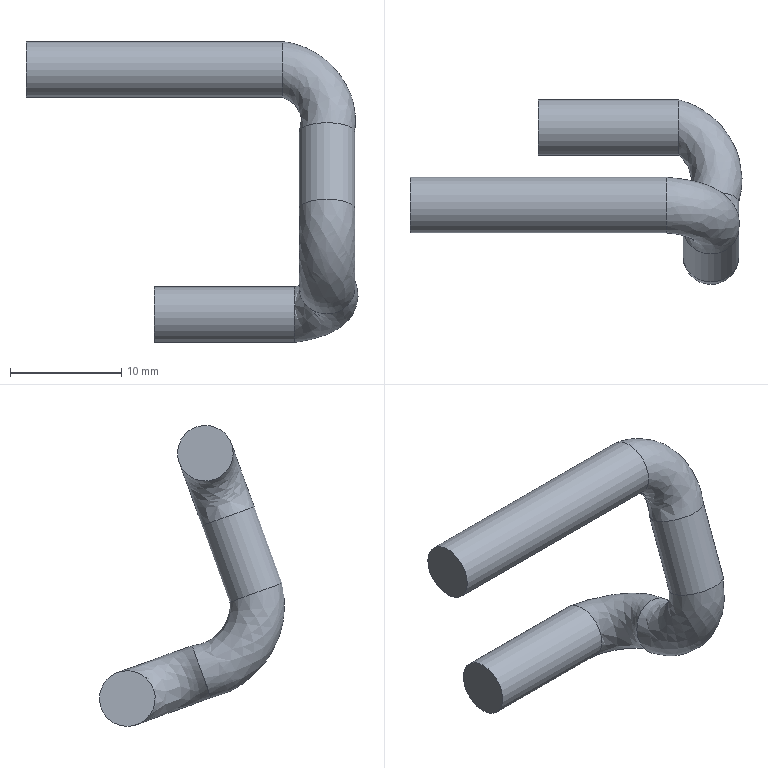Component | NX | HOSE | 2 solids | 10 faces | box 29.94 x 16.61 x 27 mm | volume 1335 mm3 | plane 4 | cylinder 3 | other 3 | commonest cylinder face diameters 5 x3
STEP:
#1=CARTESIAN_POINT('',(0.,0.,0.));
#2=DIRECTION('',(0.,0.,1.));
#3=DIRECTION('',(1.,0.,0.));
#4=AXIS2_PLACEMENT_3D('',#1,#2,#3);
#5=CARTESIAN_POINT('',(84.825,2.35,-26.852));
#6=VERTEX_POINT('',#5);
#7=CARTESIAN_POINT('',(84.825,0.,-26.));
#8=DIRECTION('',(1.,-0.,0.));
#9=DIRECTION('',(0.,0.9402,-0.3406));
#10=AXIS2_PLACEMENT_3D('',#7,#8,#9);
#11=CIRCLE('',#10,2.5);
#12=CARTESIAN_POINT('',(84.825,0.,-26.));
#13=DIRECTION('',(-1.,0.,0.));
#14=DIRECTION('',(0.,0.3406,0.9402));
#15=AXIS2_PLACEMENT_3D('',#12,#13,#14);
#16=CYLINDRICAL_SURFACE('',#15,2.5);
#17=CARTESIAN_POINT('',(7.854,0.));
#18=DIRECTION('',(-1.,0.));
#19=VECTOR('',#18,1.);
#20=LINE('',#17,#19);
#21=(GEOMETRIC_REPRESENTATION_CONTEXT(2)PARAMETRIC_REPRESENTATION_CONTEXT()REPRESENTATION_CONTEXT('',''));
#22=DEFINITIONAL_REPRESENTATION('',(#20),#21);
#23=PCURVE('',#16,#22);
#24=CARTESIAN_POINT('',(84.825,0.,-26.));
#25=DIRECTION('',(1.,-0.,0.));
#26=DIRECTION('',(0.,0.9402,-0.3406));
#27=AXIS2_PLACEMENT_3D('',#24,#25,#26);
#28=CIRCLE('',#27,2.5);
#29=CARTESIAN_POINT('',(82.75,-4.701,-24.297));
#30=DIRECTION('',(0.,-0.3406,-0.9402));
#31=AXIS1_PLACEMENT('',#29,#30);
#32=SURFACE_OF_REVOLUTION('',#28,#31);
#33=CARTESIAN_POINT('',(6.283,0.));
#34=DIRECTION('',(0.,1.));
#35=VECTOR('',#34,1.);
#36=LINE('',#33,#35);
#37=(GEOMETRIC_REPRESENTATION_CONTEXT(2)PARAMETRIC_REPRESENTATION_CONTEXT()REPRESENTATION_CONTEXT('',''));
#38=DEFINITIONAL_REPRESENTATION('',(#36),#37);
#39=PCURVE('',#32,#38);
#40=SURFACE_CURVE('',#11,(#23,#39),.PCURVE_S1.);
#41=EDGE_CURVE('',#6,#6,#40,.T.);
#42=ORIENTED_EDGE('',*,*,#41,.F.);
#43=CARTESIAN_POINT('',(72.25,2.35,-26.852));
#44=VERTEX_POINT('',#43);
#45=CARTESIAN_POINT('',(84.825,2.35,-26.852));
#46=CARTESIAN_POINT('',(72.25,2.35,-26.852));
#47=B_SPLINE_CURVE_WITH_KNOTS('',1,(#45,#46),.UNSPECIFIED.,.F.,.F.,(2,2),(0.,12.575),.PIECEWISE_BEZIER_KNOTS.);
#48=CARTESIAN_POINT('',(7.854,0.));
#49=DIRECTION('',(0.,1.));
#50=VECTOR('',#49,1.);
#51=LINE('',#48,#50);
#52=(GEOMETRIC_REPRESENTATION_CONTEXT(2)PARAMETRIC_REPRESENTATION_CONTEXT()REPRESENTATION_CONTEXT('',''));
#53=DEFINITIONAL_REPRESENTATION('',(#51),#52);
#54=PCURVE('',#16,#53);
#55=CARTESIAN_POINT('',(1.571,0.));
#56=DIRECTION('',(0.,1.));
#57=VECTOR('',#56,1.);
#58=LINE('',#55,#57);
#59=(GEOMETRIC_REPRESENTATION_CONTEXT(2)PARAMETRIC_REPRESENTATION_CONTEXT()REPRESENTATION_CONTEXT('',''));
#60=DEFINITIONAL_REPRESENTATION('',(#58),#59);
#61=PCURVE('',#16,#60);
#62=SEAM_CURVE('',#47,(#54,#61),.PCURVE_S1.);
#63=EDGE_CURVE('',#6,#44,#62,.T.);
#64=ORIENTED_EDGE('',*,*,#63,.T.);
#65=CARTESIAN_POINT('',(72.25,0.,-26.));
#66=DIRECTION('',(1.,-0.,0.));
#67=DIRECTION('',(0.,0.9402,-0.3406));
#68=AXIS2_PLACEMENT_3D('',#65,#66,#67);
#69=CIRCLE('',#68,2.5);
#70=CARTESIAN_POINT('',(7.854,12.575));
#71=DIRECTION('',(-1.,0.));
#72=VECTOR('',#71,1.);
#73=LINE('',#70,#72);
#74=(GEOMETRIC_REPRESENTATION_CONTEXT(2)PARAMETRIC_REPRESENTATION_CONTEXT()REPRESENTATION_CONTEXT('',''));
#75=DEFINITIONAL_REPRESENTATION('',(#73),#74);
#76=PCURVE('',#16,#75);
#77=CARTESIAN_POINT('',(72.25,0.,-26.));
#78=DIRECTION('',(1.,-0.,0.));
#79=DIRECTION('',(0.,-0.3406,-0.9402));
#80=AXIS2_PLACEMENT_3D('',#77,#78,#79);
#81=PLANE('',#80);
#82=CARTESIAN_POINT('',(0.,0.));
#83=DIRECTION('',(0.,1.));
#84=AXIS2_PLACEMENT_2D('',#82,#83);
#85=CIRCLE('',#84,2.5);
#86=(GEOMETRIC_REPRESENTATION_CONTEXT(2)PARAMETRIC_REPRESENTATION_CONTEXT()REPRESENTATION_CONTEXT('',''));
#87=DEFINITIONAL_REPRESENTATION('',(#85),#86);
#88=PCURVE('',#81,#87);
#89=SURFACE_CURVE('',#69,(#76,#88),.PCURVE_S1.);
#90=EDGE_CURVE('',#44,#44,#89,.T.);
#91=ORIENTED_EDGE('',*,*,#90,.T.);
#92=ORIENTED_EDGE('',*,*,#63,.F.);
#93=EDGE_LOOP('',(#42,#64,#91,#92));
#94=FACE_BOUND('',#93,.T.);
#95=ADVANCED_FACE('',(#94),#16,.T.);
#96=ORIENTED_EDGE('',*,*,#41,.F.);
#97=CARTESIAN_POINT('',(90.25,-6.652,-23.59));
#98=VERTEX_POINT('',#97);
#99=CARTESIAN_POINT('',(84.825,2.35,-26.852));
#100=CARTESIAN_POINT('',(86.83,1.829,-26.663));
#101=CARTESIAN_POINT('',(88.607,0.7215,-26.261));
#102=CARTESIAN_POINT('',(89.95,-0.8659,-25.686));
#103=CARTESIAN_POINT('',(90.708,-2.765,-24.998));
#104=CARTESIAN_POINT('',(90.805,-4.767,-24.273));
#105=CARTESIAN_POINT('',(90.25,-6.652,-23.59));
#106=(BOUNDED_CURVE()B_SPLINE_CURVE(6,(#99,#100,#101,#102,#103,#104,#105),.UNSPECIFIED.,.F.,.F.)B_SPLINE_CURVE_WITH_KNOTS((7,7),(0.,1.571),.PIECEWISE_BEZIER_KNOTS.)CURVE()GEOMETRIC_REPRESENTATION_ITEM()RATIONAL_B_SPLINE_CURVE((1.031,1.01,0.9979,0.994,0.9979,1.01,1.031))REPRESENTATION_ITEM(''));
#107=CARTESIAN_POINT('',(6.283,0.));
#108=DIRECTION('',(1.,0.));
#109=VECTOR('',#108,1.);
#110=LINE('',#107,#109);
#111=(GEOMETRIC_REPRESENTATION_CONTEXT(2)PARAMETRIC_REPRESENTATION_CONTEXT()REPRESENTATION_CONTEXT('',''));
#112=DEFINITIONAL_REPRESENTATION('',(#110),#111);
#113=PCURVE('',#32,#112);
#114=CARTESIAN_POINT('',(6.283,6.283));
#115=DIRECTION('',(1.,0.));
#116=VECTOR('',#115,1.);
#117=LINE('',#114,#116);
#118=(GEOMETRIC_REPRESENTATION_CONTEXT(2)PARAMETRIC_REPRESENTATION_CONTEXT()REPRESENTATION_CONTEXT('',''));
#119=DEFINITIONAL_REPRESENTATION('',(#117),#118);
#120=PCURVE('',#32,#119);
#121=SEAM_CURVE('',#106,(#113,#120),.PCURVE_S1.);
#122=EDGE_CURVE('',#6,#98,#121,.T.);
#123=ORIENTED_EDGE('',*,*,#122,.T.);
#124=CARTESIAN_POINT('',(87.75,-6.652,-23.59));
#125=DIRECTION('',(0.,-0.9402,0.3406));
#126=DIRECTION('',(1.,0.,0.));
#127=AXIS2_PLACEMENT_3D('',#124,#125,#126);
#128=CIRCLE('',#127,2.5);
#129=CARTESIAN_POINT('',(7.854,0.));
#130=DIRECTION('',(0.,1.));
#131=VECTOR('',#130,1.);
#132=LINE('',#129,#131);
#133=(GEOMETRIC_REPRESENTATION_CONTEXT(2)PARAMETRIC_REPRESENTATION_CONTEXT()REPRESENTATION_CONTEXT('',''));
#134=DEFINITIONAL_REPRESENTATION('',(#132),#133);
#135=PCURVE('',#32,#134);
#136=CARTESIAN_POINT('',(87.75,-6.652,-23.59));
#137=DIRECTION('',(0.,-0.9402,0.3406));
#138=DIRECTION('',(0.,-0.3406,-0.9402));
#139=AXIS2_PLACEMENT_3D('',#136,#137,#138);
#140=PLANE('',#139);
#141=CARTESIAN_POINT('',(0.,0.));
#142=DIRECTION('',(0.,1.));
#143=AXIS2_PLACEMENT_2D('',#141,#142);
#144=CIRCLE('',#143,2.5);
#145=(GEOMETRIC_REPRESENTATION_CONTEXT(2)PARAMETRIC_REPRESENTATION_CONTEXT()REPRESENTATION_CONTEXT('',''));
#146=DEFINITIONAL_REPRESENTATION('',(#144),#145);
#147=PCURVE('',#140,#146);
#148=SURFACE_CURVE('',#128,(#135,#147),.PCURVE_S1.);
#149=EDGE_CURVE('',#98,#98,#148,.T.);
#150=ORIENTED_EDGE('',*,*,#149,.T.);
#151=ORIENTED_EDGE('',*,*,#122,.F.);
#152=EDGE_LOOP('',(#96,#123,#150,#151));
#153=FACE_BOUND('',#152,.F.);
#154=ADVANCED_FACE('',(#153),#32,.F.);
#155=ORIENTED_EDGE('',*,*,#90,.F.);
#156=EDGE_LOOP('',(#155));
#157=FACE_BOUND('',#156,.T.);
#158=ADVANCED_FACE('',(#157),#81,.F.);
#159=ORIENTED_EDGE('',*,*,#149,.T.);
#160=EDGE_LOOP('',(#159));
#161=FACE_BOUND('',#160,.T.);
#162=ADVANCED_FACE('',(#161),#140,.T.);
#163=CLOSED_SHELL('',(#95,#154,#158,#162));
#164=MANIFOLD_SOLID_BREP('',#163);
#165=(LENGTH_UNIT()NAMED_UNIT(*)SI_UNIT(.MILLI.,.METRE.));
#166=UNCERTAINTY_MEASURE_WITH_UNIT(LENGTH_MEASURE(0.00001),#165,'','');
#167=(NAMED_UNIT(*)PLANE_ANGLE_UNIT()SI_UNIT($,.RADIAN.));
#168=(NAMED_UNIT(*)SI_UNIT($,.STERADIAN.)SOLID_ANGLE_UNIT());
#169=(GEOMETRIC_REPRESENTATION_CONTEXT(3)GLOBAL_UNCERTAINTY_ASSIGNED_CONTEXT((#166))GLOBAL_UNIT_ASSIGNED_CONTEXT((#165,#167,#168))REPRESENTATION_CONTEXT('',''));
#170=ADVANCED_BREP_SHAPE_REPRESENTATION('',(#4,#164),#169);
#171=CARTESIAN_POINT('',(0.,0.,0.));
#172=DIRECTION('',(0.,0.,1.));
#173=DIRECTION('',(1.,0.,0.));
#174=AXIS2_PLACEMENT_3D('',#171,#172,#173);
#175=CARTESIAN_POINT('',(0.,0.,0.));
#176=DIRECTION('',(0.,0.,1.));
#177=DIRECTION('',(1.,0.,0.));
#178=AXIS2_PLACEMENT_3D('',#175,#176,#177);
#179=(LENGTH_UNIT()NAMED_UNIT(*)SI_UNIT(.MILLI.,.METRE.));
#180=UNCERTAINTY_MEASURE_WITH_UNIT(LENGTH_MEASURE(0.00001),#179,'','');
#181=(NAMED_UNIT(*)PLANE_ANGLE_UNIT()SI_UNIT($,.RADIAN.));
#182=(NAMED_UNIT(*)SI_UNIT($,.STERADIAN.)SOLID_ANGLE_UNIT());
#183=(GEOMETRIC_REPRESENTATION_CONTEXT(3)GLOBAL_UNCERTAINTY_ASSIGNED_CONTEXT((#180))GLOBAL_UNIT_ASSIGNED_CONTEXT((#179,#181,#182))REPRESENTATION_CONTEXT('',''));
#184=SHAPE_REPRESENTATION('',(#4,#174,#178),#183);
#185=ITEM_DEFINED_TRANSFORMATION('','',#4,#174);
#186=(REPRESENTATION_RELATIONSHIP('','',#170,#184)REPRESENTATION_RELATIONSHIP_WITH_TRANSFORMATION(#185)SHAPE_REPRESENTATION_RELATIONSHIP());
#187=CARTESIAN_POINT('',(83.75,-6.148,-1.65));
#188=VERTEX_POINT('',#187);
#189=CARTESIAN_POINT('',(83.75,-7.,-4.));
#190=DIRECTION('',(-1.,-0.,0.));
#191=DIRECTION('',(0.,0.3406,0.9402));
#192=AXIS2_PLACEMENT_3D('',#189,#190,#191);
#193=CIRCLE('',#192,2.5);
#194=CARTESIAN_POINT('',(83.75,-7.,-4.));
#195=DIRECTION('',(-1.,0.,0.));
#196=DIRECTION('',(0.,0.3406,0.9402));
#197=AXIS2_PLACEMENT_3D('',#194,#195,#196);
#198=CYLINDRICAL_SURFACE('',#197,2.5);
#199=CARTESIAN_POINT('',(0.,0.));
#200=DIRECTION('',(1.,0.));
#201=VECTOR('',#200,1.);
#202=LINE('',#199,#201);
#203=(GEOMETRIC_REPRESENTATION_CONTEXT(2)PARAMETRIC_REPRESENTATION_CONTEXT()REPRESENTATION_CONTEXT('',''));
#204=DEFINITIONAL_REPRESENTATION('',(#202),#203);
#205=PCURVE('',#198,#204);
#206=CARTESIAN_POINT('',(87.75,-9.044,-9.641));
#207=DIRECTION('',(0.,0.3406,0.9402));
#208=DIRECTION('',(1.,-0.,0.));
#209=AXIS2_PLACEMENT_3D('',#206,#207,#208);
#210=CIRCLE('',#209,2.5);
#211=CARTESIAN_POINT('',(82.75,-8.703,-8.701));
#212=DIRECTION('',(0.,-0.9402,0.3406));
#213=AXIS1_PLACEMENT('',#211,#212);
#214=SURFACE_OF_REVOLUTION('',#210,#213);
#215=CARTESIAN_POINT('',(7.854,0.));
#216=DIRECTION('',(0.,1.));
#217=VECTOR('',#216,1.);
#218=LINE('',#215,#217);
#219=(GEOMETRIC_REPRESENTATION_CONTEXT(2)PARAMETRIC_REPRESENTATION_CONTEXT()REPRESENTATION_CONTEXT('',''));
#220=DEFINITIONAL_REPRESENTATION('',(#218),#219);
#221=PCURVE('',#214,#220);
#222=SURFACE_CURVE('',#193,(#205,#221),.PCURVE_S1.);
#223=EDGE_CURVE('',#188,#188,#222,.T.);
#224=ORIENTED_EDGE('',*,*,#223,.T.);
#225=CARTESIAN_POINT('',(60.75,-6.148,-1.65));
#226=VERTEX_POINT('',#225);
#227=CARTESIAN_POINT('',(83.75,-6.148,-1.65));
#228=CARTESIAN_POINT('',(60.75,-6.148,-1.65));
#229=B_SPLINE_CURVE_WITH_KNOTS('',1,(#227,#228),.UNSPECIFIED.,.F.,.F.,(2,2),(0.,23.),.PIECEWISE_BEZIER_KNOTS.);
#230=CARTESIAN_POINT('',(6.283,0.));
#231=DIRECTION('',(0.,1.));
#232=VECTOR('',#231,1.);
#233=LINE('',#230,#232);
#234=(GEOMETRIC_REPRESENTATION_CONTEXT(2)PARAMETRIC_REPRESENTATION_CONTEXT()REPRESENTATION_CONTEXT('',''));
#235=DEFINITIONAL_REPRESENTATION('',(#233),#234);
#236=PCURVE('',#198,#235);
#237=CARTESIAN_POINT('',(0.,0.));
#238=DIRECTION('',(0.,1.));
#239=VECTOR('',#238,1.);
#240=LINE('',#237,#239);
#241=(GEOMETRIC_REPRESENTATION_CONTEXT(2)PARAMETRIC_REPRESENTATION_CONTEXT()REPRESENTATION_CONTEXT('',''));
#242=DEFINITIONAL_REPRESENTATION('',(#240),#241);
#243=PCURVE('',#198,#242);
#244=SEAM_CURVE('',#229,(#236,#243),.PCURVE_S1.);
#245=EDGE_CURVE('',#188,#226,#244,.T.);
#246=ORIENTED_EDGE('',*,*,#245,.T.);
#247=CARTESIAN_POINT('',(60.75,-7.,-4.));
#248=DIRECTION('',(-1.,-0.,0.));
#249=DIRECTION('',(0.,0.3406,0.9402));
#250=AXIS2_PLACEMENT_3D('',#247,#248,#249);
#251=CIRCLE('',#250,2.5);
#252=CARTESIAN_POINT('',(0.,23.));
#253=DIRECTION('',(1.,0.));
#254=VECTOR('',#253,1.);
#255=LINE('',#252,#254);
#256=(GEOMETRIC_REPRESENTATION_CONTEXT(2)PARAMETRIC_REPRESENTATION_CONTEXT()REPRESENTATION_CONTEXT('',''));
#257=DEFINITIONAL_REPRESENTATION('',(#255),#256);
#258=PCURVE('',#198,#257);
#259=CARTESIAN_POINT('',(60.75,-7.,-4.));
#260=DIRECTION('',(-1.,-0.,0.));
#261=DIRECTION('',(0.,-0.9402,0.3406));
#262=AXIS2_PLACEMENT_3D('',#259,#260,#261);
#263=PLANE('',#262);
#264=CARTESIAN_POINT('',(0.,0.));
#265=DIRECTION('',(0.,1.));
#266=AXIS2_PLACEMENT_2D('',#264,#265);
#267=CIRCLE('',#266,2.5);
#268=(GEOMETRIC_REPRESENTATION_CONTEXT(2)PARAMETRIC_REPRESENTATION_CONTEXT()REPRESENTATION_CONTEXT('',''));
#269=DEFINITIONAL_REPRESENTATION('',(#267),#268);
#270=PCURVE('',#263,#269);
#271=SURFACE_CURVE('',#251,(#258,#270),.PCURVE_S1.);
#272=EDGE_CURVE('',#226,#226,#271,.T.);
#273=ORIENTED_EDGE('',*,*,#272,.F.);
#274=ORIENTED_EDGE('',*,*,#245,.F.);
#275=EDGE_LOOP('',(#224,#246,#273,#274));
#276=FACE_BOUND('',#275,.T.);
#277=ADVANCED_FACE('',(#276),#198,.T.);
#278=CARTESIAN_POINT('',(90.25,-9.044,-9.641));
#279=VERTEX_POINT('',#278);
#280=CARTESIAN_POINT('',(87.75,-9.044,-9.641));
#281=DIRECTION('',(0.,0.3406,0.9402));
#282=DIRECTION('',(1.,0.,0.));
#283=AXIS2_PLACEMENT_3D('',#280,#281,#282);
#284=CIRCLE('',#283,2.5);
#285=CARTESIAN_POINT('',(6.283,0.));
#286=DIRECTION('',(0.,1.));
#287=VECTOR('',#286,1.);
#288=LINE('',#285,#287);
#289=(GEOMETRIC_REPRESENTATION_CONTEXT(2)PARAMETRIC_REPRESENTATION_CONTEXT()REPRESENTATION_CONTEXT('',''));
#290=DEFINITIONAL_REPRESENTATION('',(#288),#289);
#291=PCURVE('',#214,#290);
#292=CARTESIAN_POINT('',(87.75,-11.53,-16.505));
#293=DIRECTION('',(0.,0.3406,0.9402));
#294=DIRECTION('',(1.,0.,0.));
#295=AXIS2_PLACEMENT_3D('',#292,#293,#294);
#296=CYLINDRICAL_SURFACE('',#295,2.5);
#297=CARTESIAN_POINT('',(0.,7.3));
#298=DIRECTION('',(1.,0.));
#299=VECTOR('',#298,1.);
#300=LINE('',#297,#299);
#301=(GEOMETRIC_REPRESENTATION_CONTEXT(2)PARAMETRIC_REPRESENTATION_CONTEXT()REPRESENTATION_CONTEXT('',''));
#302=DEFINITIONAL_REPRESENTATION('',(#300),#301);
#303=PCURVE('',#296,#302);
#304=SURFACE_CURVE('',#284,(#291,#303),.PCURVE_S1.);
#305=EDGE_CURVE('',#279,#279,#304,.T.);
#306=ORIENTED_EDGE('',*,*,#305,.F.);
#307=CARTESIAN_POINT('',(90.25,-9.044,-9.641));
#308=CARTESIAN_POINT('',(90.517,-8.361,-7.756));
#309=CARTESIAN_POINT('',(90.14,-7.667,-5.84));
#310=CARTESIAN_POINT('',(89.141,-7.038,-4.106));
#311=CARTESIAN_POINT('',(87.623,-6.545,-2.745));
#312=CARTESIAN_POINT('',(85.755,-6.239,-1.901));
#313=CARTESIAN_POINT('',(83.75,-6.148,-1.65));
#314=(BOUNDED_CURVE()B_SPLINE_CURVE(6,(#307,#308,#309,#310,#311,#312,#313),.UNSPECIFIED.,.F.,.F.)B_SPLINE_CURVE_WITH_KNOTS((7,7),(0.,1.571),.PIECEWISE_BEZIER_KNOTS.)CURVE()GEOMETRIC_REPRESENTATION_ITEM()RATIONAL_B_SPLINE_CURVE((1.031,1.01,0.9979,0.994,0.9979,1.01,1.031))REPRESENTATION_ITEM(''));
#315=CARTESIAN_POINT('',(6.283,0.));
#316=DIRECTION('',(1.,0.));
#317=VECTOR('',#316,1.);
#318=LINE('',#315,#317);
#319=(GEOMETRIC_REPRESENTATION_CONTEXT(2)PARAMETRIC_REPRESENTATION_CONTEXT()REPRESENTATION_CONTEXT('',''));
#320=DEFINITIONAL_REPRESENTATION('',(#318),#319);
#321=PCURVE('',#214,#320);
#322=CARTESIAN_POINT('',(6.283,6.283));
#323=DIRECTION('',(1.,0.));
#324=VECTOR('',#323,1.);
#325=LINE('',#322,#324);
#326=(GEOMETRIC_REPRESENTATION_CONTEXT(2)PARAMETRIC_REPRESENTATION_CONTEXT()REPRESENTATION_CONTEXT('',''));
#327=DEFINITIONAL_REPRESENTATION('',(#325),#326);
#328=PCURVE('',#214,#327);
#329=SEAM_CURVE('',#314,(#321,#328),.PCURVE_S1.);
#330=EDGE_CURVE('',#279,#188,#329,.T.);
#331=ORIENTED_EDGE('',*,*,#330,.T.);
#332=ORIENTED_EDGE('',*,*,#223,.T.);
#333=ORIENTED_EDGE('',*,*,#330,.F.);
#334=EDGE_LOOP('',(#306,#331,#332,#333));
#335=FACE_BOUND('',#334,.F.);
#336=ADVANCED_FACE('',(#335),#214,.F.);
#337=CARTESIAN_POINT('',(90.25,-11.53,-16.505));
#338=VERTEX_POINT('',#337);
#339=CARTESIAN_POINT('',(87.75,-11.53,-16.505));
#340=DIRECTION('',(0.,0.3406,0.9402));
#341=DIRECTION('',(1.,0.,0.));
#342=AXIS2_PLACEMENT_3D('',#339,#340,#341);
#343=CIRCLE('',#342,2.5);
#344=CARTESIAN_POINT('',(0.,0.));
#345=DIRECTION('',(1.,0.));
#346=VECTOR('',#345,1.);
#347=LINE('',#344,#346);
#348=(GEOMETRIC_REPRESENTATION_CONTEXT(2)PARAMETRIC_REPRESENTATION_CONTEXT()REPRESENTATION_CONTEXT('',''));
#349=DEFINITIONAL_REPRESENTATION('',(#347),#348);
#350=PCURVE('',#296,#349);
#351=CARTESIAN_POINT('',(87.75,-11.53,-16.505));
#352=DIRECTION('',(0.,0.3406,0.9402));
#353=DIRECTION('',(1.,-0.,0.));
#354=AXIS2_PLACEMENT_3D('',#351,#352,#353);
#355=CIRCLE('',#354,2.5);
#356=CARTESIAN_POINT('',(87.75,-5.549,-17.608));
#357=DIRECTION('',(1.,0.,0.));
#358=AXIS1_PLACEMENT('',#356,#357);
#359=SURFACE_OF_REVOLUTION('',#355,#358);
#360=CARTESIAN_POINT('',(6.283,0.));
#361=DIRECTION('',(0.,1.));
#362=VECTOR('',#361,1.);
#363=LINE('',#360,#362);
#364=(GEOMETRIC_REPRESENTATION_CONTEXT(2)PARAMETRIC_REPRESENTATION_CONTEXT()REPRESENTATION_CONTEXT('',''));
#365=DEFINITIONAL_REPRESENTATION('',(#363),#364);
#366=PCURVE('',#359,#365);
#367=SURFACE_CURVE('',#343,(#350,#366),.PCURVE_S1.);
#368=EDGE_CURVE('',#338,#338,#367,.T.);
#369=ORIENTED_EDGE('',*,*,#368,.T.);
#370=CARTESIAN_POINT('',(90.25,-11.53,-16.505));
#371=CARTESIAN_POINT('',(90.25,-9.044,-9.641));
#372=B_SPLINE_CURVE_WITH_KNOTS('',1,(#370,#371),.UNSPECIFIED.,.F.,.F.,(2,2),(0.,7.3),.PIECEWISE_BEZIER_KNOTS.);
#373=CARTESIAN_POINT('',(6.283,0.));
#374=DIRECTION('',(0.,1.));
#375=VECTOR('',#374,1.);
#376=LINE('',#373,#375);
#377=(GEOMETRIC_REPRESENTATION_CONTEXT(2)PARAMETRIC_REPRESENTATION_CONTEXT()REPRESENTATION_CONTEXT('',''));
#378=DEFINITIONAL_REPRESENTATION('',(#376),#377);
#379=PCURVE('',#296,#378);
#380=CARTESIAN_POINT('',(0.,0.));
#381=DIRECTION('',(0.,1.));
#382=VECTOR('',#381,1.);
#383=LINE('',#380,#382);
#384=(GEOMETRIC_REPRESENTATION_CONTEXT(2)PARAMETRIC_REPRESENTATION_CONTEXT()REPRESENTATION_CONTEXT('',''));
#385=DEFINITIONAL_REPRESENTATION('',(#383),#384);
#386=PCURVE('',#296,#385);
#387=SEAM_CURVE('',#372,(#379,#386),.PCURVE_S1.);
#388=EDGE_CURVE('',#338,#279,#387,.T.);
#389=ORIENTED_EDGE('',*,*,#388,.T.);
#390=ORIENTED_EDGE('',*,*,#305,.F.);
#391=ORIENTED_EDGE('',*,*,#388,.F.);
#392=EDGE_LOOP('',(#369,#389,#390,#391));
#393=FACE_BOUND('',#392,.T.);
#394=ADVANCED_FACE('',(#393),#296,.T.);
#395=ORIENTED_EDGE('',*,*,#368,.F.);
#396=CARTESIAN_POINT('',(90.25,-6.652,-23.59));
#397=VERTEX_POINT('',#396);
#398=CARTESIAN_POINT('',(90.25,-11.53,-16.505));
#399=CARTESIAN_POINT('',(90.25,-11.825,-18.104));
#400=CARTESIAN_POINT('',(90.25,-11.604,-19.755));
#401=CARTESIAN_POINT('',(90.25,-10.876,-21.276));
#402=CARTESIAN_POINT('',(90.25,-9.715,-22.499));
#403=CARTESIAN_POINT('',(90.25,-8.251,-23.295));
#404=CARTESIAN_POINT('',(90.25,-6.652,-23.59));
#405=(BOUNDED_CURVE()B_SPLINE_CURVE(6,(#398,#399,#400,#401,#402,#403,#404),.UNSPECIFIED.,.F.,.F.)B_SPLINE_CURVE_WITH_KNOTS((7,7),(0.,1.571),.PIECEWISE_BEZIER_KNOTS.)CURVE()GEOMETRIC_REPRESENTATION_ITEM()RATIONAL_B_SPLINE_CURVE((1.031,1.01,0.9979,0.994,0.9979,1.01,1.031))REPRESENTATION_ITEM(''));
#406=CARTESIAN_POINT('',(6.283,0.));
#407=DIRECTION('',(1.,0.));
#408=VECTOR('',#407,1.);
#409=LINE('',#406,#408);
#410=(GEOMETRIC_REPRESENTATION_CONTEXT(2)PARAMETRIC_REPRESENTATION_CONTEXT()REPRESENTATION_CONTEXT('',''));
#411=DEFINITIONAL_REPRESENTATION('',(#409),#410);
#412=PCURVE('',#359,#411);
#413=CARTESIAN_POINT('',(6.283,6.283));
#414=DIRECTION('',(1.,0.));
#415=VECTOR('',#414,1.);
#416=LINE('',#413,#415);
#417=(GEOMETRIC_REPRESENTATION_CONTEXT(2)PARAMETRIC_REPRESENTATION_CONTEXT()REPRESENTATION_CONTEXT('',''));
#418=DEFINITIONAL_REPRESENTATION('',(#416),#417);
#419=PCURVE('',#359,#418);
#420=SEAM_CURVE('',#405,(#412,#419),.PCURVE_S1.);
#421=EDGE_CURVE('',#338,#397,#420,.T.);
#422=ORIENTED_EDGE('',*,*,#421,.T.);
#423=CARTESIAN_POINT('',(87.75,-6.652,-23.59));
#424=DIRECTION('',(0.,-0.9402,0.3406));
#425=DIRECTION('',(1.,0.,0.));
#426=AXIS2_PLACEMENT_3D('',#423,#424,#425);
#427=CIRCLE('',#426,2.5);
#428=CARTESIAN_POINT('',(7.854,0.));
#429=DIRECTION('',(0.,1.));
#430=VECTOR('',#429,1.);
#431=LINE('',#428,#430);
#432=(GEOMETRIC_REPRESENTATION_CONTEXT(2)PARAMETRIC_REPRESENTATION_CONTEXT()REPRESENTATION_CONTEXT('',''));
#433=DEFINITIONAL_REPRESENTATION('',(#431),#432);
#434=PCURVE('',#359,#433);
#435=CARTESIAN_POINT('',(87.75,-6.652,-23.59));
#436=DIRECTION('',(0.,-0.9402,0.3406));
#437=DIRECTION('',(0.,-0.3406,-0.9402));
#438=AXIS2_PLACEMENT_3D('',#435,#436,#437);
#439=PLANE('',#438);
#440=CARTESIAN_POINT('',(0.,0.));
#441=DIRECTION('',(0.,1.));
#442=AXIS2_PLACEMENT_2D('',#440,#441);
#443=CIRCLE('',#442,2.5);
#444=(GEOMETRIC_REPRESENTATION_CONTEXT(2)PARAMETRIC_REPRESENTATION_CONTEXT()REPRESENTATION_CONTEXT('',''));
#445=DEFINITIONAL_REPRESENTATION('',(#443),#444);
#446=PCURVE('',#439,#445);
#447=SURFACE_CURVE('',#427,(#434,#446),.PCURVE_S1.);
#448=EDGE_CURVE('',#397,#397,#447,.T.);
#449=ORIENTED_EDGE('',*,*,#448,.T.);
#450=ORIENTED_EDGE('',*,*,#421,.F.);
#451=EDGE_LOOP('',(#395,#422,#449,#450));
#452=FACE_BOUND('',#451,.T.);
#453=ADVANCED_FACE('',(#452),#359,.T.);
#454=ORIENTED_EDGE('',*,*,#272,.T.);
#455=EDGE_LOOP('',(#454));
#456=FACE_BOUND('',#455,.T.);
#457=ADVANCED_FACE('',(#456),#263,.T.);
#458=ORIENTED_EDGE('',*,*,#448,.F.);
#459=EDGE_LOOP('',(#458));
#460=FACE_BOUND('',#459,.T.);
#461=ADVANCED_FACE('',(#460),#439,.F.);
#462=CLOSED_SHELL('',(#277,#336,#394,#453,#457,#461));
#463=MANIFOLD_SOLID_BREP('',#462);
#464=(LENGTH_UNIT()NAMED_UNIT(*)SI_UNIT(.MILLI.,.METRE.));
#465=UNCERTAINTY_MEASURE_WITH_UNIT(LENGTH_MEASURE(0.00001),#464,'','');
#466=(NAMED_UNIT(*)PLANE_ANGLE_UNIT()SI_UNIT($,.RADIAN.));
#467=(NAMED_UNIT(*)SI_UNIT($,.STERADIAN.)SOLID_ANGLE_UNIT());
#468=(GEOMETRIC_REPRESENTATION_CONTEXT(3)GLOBAL_UNCERTAINTY_ASSIGNED_CONTEXT((#465))GLOBAL_UNIT_ASSIGNED_CONTEXT((#464,#466,#467))REPRESENTATION_CONTEXT('',''));
#469=ADVANCED_BREP_SHAPE_REPRESENTATION('',(#4,#463),#468);
#470=ITEM_DEFINED_TRANSFORMATION('','',#4,#178);
#471=(REPRESENTATION_RELATIONSHIP('','',#469,#184)REPRESENTATION_RELATIONSHIP_WITH_TRANSFORMATION(#470)SHAPE_REPRESENTATION_RELATIONSHIP());